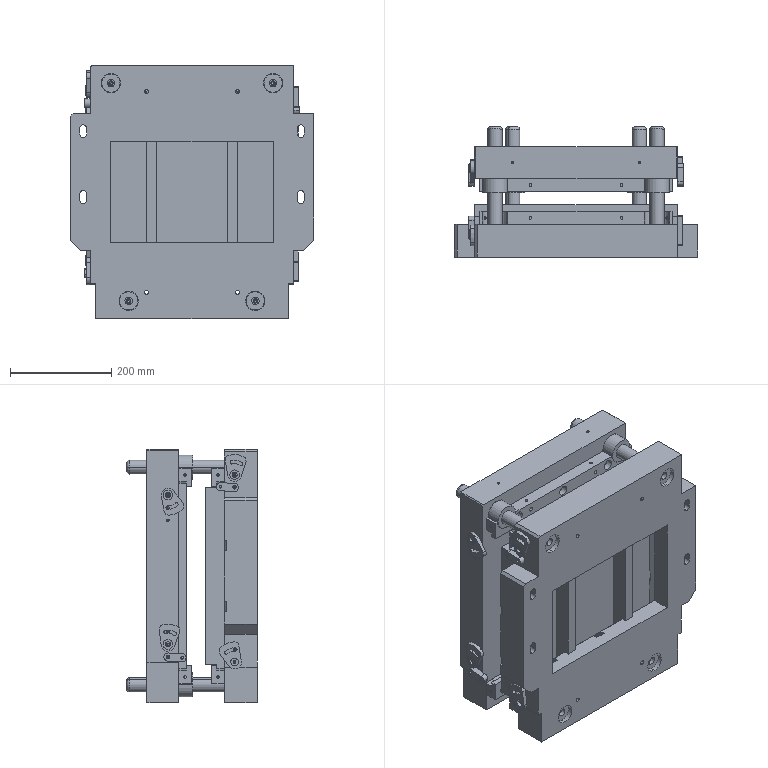Assembly | SolidWorks | mm | 38 component files | 38 solids | 988 faces | box 480 x 258 x 500 mm | volume 30255703 mm3 | cylinder 475 | plane 363 | cone 90 | torus 60 | commonest cylinder face diameters 5 x86 20 x44 48 x40 13.5 x36 8 x36 28 x32 38 x24 6.6 x24
Bill of materials:
MoldStopBlock001 | 4 |  | Flat plate with a tapered, rounded teardrop/trapezoid outline, one round through-hole near the narrow end and a curved arc slot near the wide end.
AdditionalStop | 3 |  | Thick block with a stadium/obround outline (link-like) and two round through-holes, one near each rounded end; one hole looks slightly larger than the other. A small step runs across the mid-length of one face.
GuideSlot1-01 | 2 |  | Long rectangular bar with two large semicircular saddle cutouts on the top edge near each end, a row of through-holes across the side face, small holes on the top face, and stepped/notched end blocks.
GuideSlot1 | 2 |  | Long rectangular bar with a stepped (rabbeted) L-shaped cross-section, two semicircular cutouts open to the bottom edge, and a row of through-holes in the side face. It looks like a counterpart to a similar saddle bar.
LocatingPin | 2 |  | Plain solid cylindrical rod with one end rounded/domed and the other end apparently flat.
GuidePin | 4 |  | Slender cylindrical pin with a thin integral collar near one end, a short stub past the collar, a small axial center hole/recess in the stub end, and a slightly rounded or chamfered opposite end.
LowerDieSet | 1 |  | Thick rectangular frame plate with a large central rectangular opening, stepped side tabs, chamfered corners, large corner holes, small holes, slotted holes on the side tabs, and small holes and notches on the edges.
MoldPlate | 1 |  | Plain rectangular plate with a small step or lip along two opposite edges, giving a slightly offset or rabbeted edge profile.
MoldSlotBaffle | 4 |  | Rectangular block or plate with four chamfered corners and two round through-holes lined up along one side of the face.
PinDiameter15 | 3 |  | Flanged cylindrical bushing: a thin wide flange on one end of a cylindrical body, with a straight central through-bore.
ReinforcingRib001 | 2 |  | Long narrow flat bar with chamfered corners at both ends and two small through-holes near the ends; the cross-section has bevelled long edges.
SpacerBlock | 4 |  | Stepped annular washer/spacer: a wider disc with a smaller-diameter raised boss on one side and a central through-hole.
GuideBushing | 4 |  | Hollow cylindrical sleeve (thick-walled tube) with a concentric through-bore and three narrow, round-bottomed circumferential grooves grouped near one end of the outer surface; the remaining length is plain.
KF525R2-MJ-A001 | 1 | 55 | Thick rectangular plate with a step: one end section is slightly narrower than the main body. It has four large through-holes near the corners, several small holes on the main face near each end, and small holes on the edge faces.
MoldUpperPlate510x280 | 1 |  | Plain thin rectangular plate or block with flat parallel faces and no visible holes, cutouts, or edge features.
Mates:
1. concentric | PinDiameter15-1 face at (-266.846, -14.073, 553) dir (1, 0, 0) r 7.5 | MoldStopBlock001-1 face at (-264.896, -14.073, 553) dir (1, 0, 0) r 7.5
2. coincident | PinDiameter15-1 face at (-264.896, -14.073, 553) dir (1, 0, 0) | MoldStopBlock001-1 face at (-264.896, -14.073, 553) dir (-1, 0, 0)
3. concentric | NewDieSet-1/LowerDieSetAssembly-1/LowerDieSet-1 face at (-256.746, -14.073, 553) dir (-1, 0, 0) r 2.5 | PinDiameter15-1 face at (-266.846, -14.073, 553) dir (-1, 0, 0) r 2.65
4. coincident | NewDieSet-1/LowerDieSetAssembly-1/LowerDieSet-1 face at (-256.746, -59.073, 603) dir (-1, 0, 0) | PinDiameter15-1 face at (-256.746, -14.073, 553) dir (1, 0, 0)
5. parallel | LowerDieSetAssembly-1/LowerDieSet-1 face at (329.721, -20.659, 572.489) dir (0, 1, 0) | UpperDieSetAssembly-1/KF525R2-MJ-A001-1 face at (-70.279, 69.341, 572.489) dir (0, -1, 0)
6. concentric | LowerDieSetAssembly-1/LowerDieSet-1 face at (254.721, -70.659, 107.489) dir (0, -1, 0) r 19 | SpacerBlock-1 face at (254.721, -77.659, 107.489) dir (0, 1, 0) r 18
7. coincident | SpacerBlock-2 face at (4.721, -77.659, 107.489) dir (0, -1, 0) | SpacerBlock-3 face at (-30.279, -77.659, 537.489) dir (0, -1, 0)
8. coincident | SpacerBlock-3 face at (-30.279, -77.659, 537.489) dir (0, -1, 0) | SpacerBlock-4 face at (289.721, -77.659, 537.489) dir (0, -1, 0)
9. coincident | SpacerBlock-1 face at (254.721, -77.659, 107.489) dir (0, -1, 0) | SpacerBlock-4 face at (289.721, -77.659, 537.489) dir (0, -1, 0)
10. coincident | LowerDieSetAssembly-1/LowerDieSet-1 face at (254.721, -70.659, 107.489) dir (0, -1, 0) | SpacerBlock-1 face at (254.721, -70.659, 107.489) dir (0, 1, 0)
11. concentric | LowerDieSetAssembly-1/LowerDieSet-1 face at (-30.279, -70.659, 537.489) dir (0, -1, 0) r 19 | SpacerBlock-3 face at (-30.279, -77.659, 537.489) dir (0, 1, 0) r 18
12. concentric | NewDieSet face at (59.721, 111.341, 32.489) dir (0, -1, 0) r 4 | LocatingPin-1 face at (39.721, 4.341, 520.589) dir (0, -1, 0) r 4
13. distance | LocatingPin-1 face at (39.721, 4.341, 520.589) dir (0, 1, 0) | NewDieSet face at (-0.2789, -20.659, 42.189) dir (0, -1, 0)
14. concentric | NewDieSet face at (139.721, 111.341, 32.489) dir (0, -1, 0) r 4 | LocatingPin-2 face at (219.721, 4.341, 520.589) dir (0, -1, 0) r 4
15. distance | NewDieSet face at (-0.2789, -20.659, 42.189) dir (0, -1, 0) | LocatingPin-2 face at (219.721, -35.659, 520.589) dir (0, -1, 0)
16. parallel | LowerDieSetAssembly-1/LowerDieSet-1 face at (329.721, -85.659, 572.489) dir (0, -1, 0) | NewDieSet plane at (0, 0, 0) dir (0, 1, 0)
17. concentric | LowerDieSetAssembly-1/GuidePin-4 face at (289.721, -47.659, 537.489) dir (0, -1, 0) r 3.4 | SpacerBlock-4 face at (289.721, -77.659, 537.489) dir (0, -1, 0) r 7.5
18. concentric | LowerDieSetAssembly-1/LowerDieSet-1 edge at (4.721, -70.659, 107.489) dir (0, -1, 0) r 19 | SpacerBlock-2 face at (4.721, -77.659, 107.489) dir (0, -1, 0) r 7.5
19. coincident | LocatingPin-1 face at (39.721, 4.341, 520.589) dir (0, 1, 0) | LocatingPin-2 face at (219.721, 4.341, 520.589) dir (0, 1, 0)
20. distance | LocatingPin-1 face at (39.721, -35.659, 520.589) dir (0, -1, 0) | LowerDieSetAssembly-1/LowerDieSet-1 face at (329.721, -20.659, 572.489) dir (0, 1, 0)
21. coincident | LowerDieSetAssembly-1/LowerDieSet-1 face at (329.721, -20.659, 572.489) dir (0, 1, 0) | GuideSlot1-01-4 face at (319.721, -20.659, 505.589) dir (0, -1, 0)
22. parallel | LowerDieSetAssembly-1/LowerDieSet-1 face at (329.721, -85.659, 572.489) dir (0, 0, 1) | GuideSlot1-01-4 face at (319.721, 4.441, 505.589) dir (0, 0, -1)
23. width | GuideSlot1-01-4 face at (-60.279, 4.441, 505.589) dir (-1, 0, 0) | GuideSlot1-01-4 face at (319.721, 4.441, 505.589) dir (1, 0, 0) | LowerDieSetAssembly-1/LowerDieSet-1 face at (-70.279, -85.659, 572.489) dir (-1, 0, 0) | LowerDieSetAssembly-1/LowerDieSet-1 face at (329.721, -85.659, 572.489) dir (1, 0, 0)
24. concentric | LowerDieSetAssembly-1/GuidePin-3 face at (-30.279, -47.659, 537.489) dir (0, 1, 0) r 14 | UpperDieSetAssembly-1/GuideBushing-1 face at (-30.279, 132.341, 537.489) dir (0, -1, 0) r 14
25. concentric | LowerDieSetAssembly-1/GuidePin-1 face at (254.721, -47.659, 107.489) dir (0, 1, 0) r 14 | UpperDieSetAssembly-1/GuideBushing-3 face at (254.721, 132.341, 107.489) dir (0, -1, 0) r 14
26. distance | UpperDieSetAssembly-1/KF525R2-MJ-A001-1 face at (-70.279, 69.341, 572.489) dir (0, -1, 0) | LowerDieSetAssembly-1/LowerDieSet-1 face at (329.721, -20.659, 572.489) dir (0, 1, 0)
27. concentric | LocatingPin-1 face at (39.721, 4.341, 520.589) dir (0, -1, 0) r 4 | GuideSlot1-01-4 face at (39.721, 111.341, 520.589) dir (0, -1, 0) r 4
28. concentric | LocatingPin-2 face at (219.721, 4.341, 520.589) dir (0, -1, 0) r 4 | GuideSlot1-01-4 face at (219.721, 111.341, 520.589) dir (0, -1, 0) r 4
29. parallel | LowerDieSetAssembly-1/LowerDieSet-1 face at (329.721, -85.659, 72.489) dir (0, 0, -1) | GuideSlot1-2 face at (-60.279, 4.441, 139.389) dir (0, 0, 1)
30. coincident | LowerDieSetAssembly-1/LowerDieSet-1 face at (329.721, -20.659, 572.489) dir (0, 1, 0) | GuideSlot1-2 face at (-60.279, -20.659, 139.389) dir (0, -1, 0)
31. coincident | LowerDieSetAssembly-1/LowerDieSet-1 face at (39.721, -59.659, 172.489) dir (1, 0, 0) | ReinforcingRib001-2 face at (39.721, -59.659, 472.489) dir (-1, 0, 0)
32. coincident | LowerDieSetAssembly-1/LowerDieSet-1 face at (59.721, -59.659, 472.489) dir (0, 0, -1) | ReinforcingRib001-2 face at (49.721, -40.159, 472.489) dir (0, 0, 1)
33. coincident | LowerDieSetAssembly-1/LowerDieSet-1 face at (329.721, -20.659, 572.489) dir (0, 1, 0) | ReinforcingRib001-2 face at (39.721, -20.659, 472.489) dir (0, 1, 0)
34. coincident | LowerDieSetAssembly-1/LowerDieSet-1 face at (329.721, -20.659, 572.489) dir (0, 1, 0) | ReinforcingRib001-1 face at (199.721, -20.659, 472.489) dir (0, 1, 0)
35. coincident | UpperDieSetAssembly-1/KF525R2-MJ-A001-1 face at (-70.279, 69.341, 572.489) dir (0, -1, 0) | GuideSlot1-01-5 face at (-60.279, 69.341, 505.589) dir (0, 1, 0)
36. coincident | UpperDieSetAssembly-1/KF525R2-MJ-A001-1 face at (-70.279, 69.341, 572.489) dir (0, -1, 0) | GuideSlot1-4 face at (319.721, 69.341, 139.389) dir (0, 1, 0)
37. concentric | UpperDieSetAssembly-1/KF525R2-MJ-A001-1 face at (294.721, 69.341, 124.389) dir (0, -1, 0) r 5.1 | GuideSlot1-4 face at (294.721, 44.241, 124.389) dir (0, -1, 0) r 10
38. concentric | UpperDieSetAssembly-1/KF525R2-MJ-A001-1 face at (-35.279, 69.341, 124.389) dir (0, -1, 0) r 5.1 | GuideSlot1-4 face at (-35.279, 44.241, 124.389) dir (0, -1, 0) r 10
39. parallel | UpperDieSetAssembly-1/KF525R2-MJ-A001-1 face at (-70.279, 132.341, 572.489) dir (0, 1, 0) | MoldSlotBaffle-6 face at (329.721, 54.341, 219.989) dir (0, -1, 0)
40. concentric | UpperDieSetAssembly-1/KF525R2-MJ-A001-1 face at (329.721, 90.841, 212.489) dir (1, 0, 0) r 2.5 | MoldSlotBaffle-6 face at (329.721, 90.841, 212.489) dir (-1, 0, 0) r 3.3
41. coincident | UpperDieSetAssembly-1/KF525R2-MJ-A001-1 face at (329.721, 132.341, 572.489) dir (1, 0, 0) | MoldSlotBaffle-6 face at (329.721, 54.341, 219.989) dir (-1, 0, 0)
42. parallel | LowerDieSetAssembly-1/LowerDieSet-1 face at (329.721, -40.659, 177.489) dir (1, 0, 0) r 2.5 | MoldSlotBaffle-7 face at (339.721, -40.659, 177.489) dir (1, 0, 0) r 3.3
43. coincident | LowerDieSetAssembly-1/LowerDieSet-1 face at (329.721, -85.659, 572.489) dir (1, 0, 0) | MoldSlotBaffle-7 face at (329.721, -4.159, 184.989) dir (-1, 0, 0)
44. concentric | LowerDieSetAssembly-1/LowerDieSet-1 face at (329.721, -40.659, 177.489) dir (1, 0, 0) r 2.5 | MoldSlotBaffle-7 face at (339.721, -40.659, 177.489) dir (1, 0, 0) r 3.3
45. concentric | UpperDieSetAssembly-1/KF525R2-MJ-A001-1 face at (329.721, 90.841, 457.489) dir (1, 0, 0) r 2.5 | MoldSlotBaffle-8 face at (329.721, 90.841, 457.489) dir (-1, 0, 0) r 3.3
46. coincident | UpperDieSetAssembly-1/KF525R2-MJ-A001-1 face at (329.721, 132.341, 572.489) dir (1, 0, 0) | MoldSlotBaffle-8 face at (329.721, 54.341, 464.989) dir (-1, 0, 0)
47. concentric | UpperDieSetAssembly-1/KF525R2-MJ-A001-1 face at (329.721, 90.841, 432.489) dir (1, 0, 0) r 2.5 | MoldSlotBaffle-8 face at (329.721, 90.841, 432.489) dir (-1, 0, 0) r 3.3
48. coincident | UpperDieSetAssembly-1/KF525R2-MJ-A001-1 face at (-70.279, 132.341, 572.489) dir (-1, 0, 0) | MoldStopBlock001-1 face at (-70.279, 90.841, 187.489) dir (1, 0, 0)
49. coincident | UpperDieSetAssembly-1/KF525R2-MJ-A001-1 face at (-70.279, 132.341, 572.489) dir (-1, 0, 0) | PinDiameter15-3 face at (-70.279, 90.841, 187.489) dir (1, 0, 0)
50. concentric | UpperDieSetAssembly-1/KF525R2-MJ-A001-1 face at (-70.279, 90.841, 482.489) dir (-1, 0, 0) r 2.5 | MoldStopBlock001-6 face at (-78.279, 90.841, 482.489) dir (1, 0, 0) r 7.5
51. coincident | UpperDieSetAssembly-1/KF525R2-MJ-A001-1 face at (-70.279, 132.341, 572.489) dir (-1, 0, 0) | MoldStopBlock001-6 face at (-70.279, 90.841, 482.489) dir (1, 0, 0)
52. concentric | MoldStopBlock001-6 face at (-78.279, 90.841, 482.489) dir (1, 0, 0) r 7.5 | PinDiameter15-5 face at (-80.379, 90.841, 482.489) dir (1, 0, 0) r 7.5
53. coincident | UpperDieSetAssembly-1/KF525R2-MJ-A001-1 face at (-70.279, 132.341, 572.489) dir (-1, 0, 0) | PinDiameter15-5 face at (-70.279, 90.841, 482.489) dir (1, 0, 0)
54. concentric | MoldStopBlock001-1 face at (-78.279, 90.841, 187.489) dir (1, 0, 0) r 7.5 | PinDiameter15-3 face at (-80.379, 90.841, 187.489) dir (-1, 0, 0) r 2.65
55. concentric | UpperDieSetAssembly-1/KF525R2-MJ-A001-1 face at (-70.279, 90.841, 187.489) dir (-1, 0, 0) r 2.5 | PinDiameter15-3 face at (-80.379, 90.841, 187.489) dir (-1, 0, 0) r 2.65
56. concentric | LowerDieSetAssembly-1/LowerDieSet-1 face at (254.721, -20.659, 520.589) dir (0, 1, 0) r 5.1 | GuideSlot1-01-4 face at (254.721, 4.441, 520.589) dir (0, 1, 0) r 10
57. concentric | LowerDieSetAssembly-1/LowerDieSet-1 face at (-70.279, -40.659, 152.489) dir (-1, 0, 0) r 2.5 | MoldStopBlock001-7 face at (-78.279, -40.659, 152.489) dir (1, 0, 0) r 7.5
58. coincident | LowerDieSetAssembly-1/LowerDieSet-1 face at (-70.279, -85.659, 572.489) dir (-1, 0, 0) | MoldStopBlock001-7 face at (-70.279, -40.659, 152.489) dir (1, 0, 0)
59. concentric | LowerDieSetAssembly-1/LowerDieSet-1 face at (329.721, -40.659, 497.489) dir (1, 0, 0) r 2.5 | MoldSlotBaffle-9 face at (339.721, -40.659, 497.489) dir (1, 0, 0) r 3.3
60. concentric | LowerDieSetAssembly-1/LowerDieSet-1 face at (329.721, -40.659, 522.489) dir (1, 0, 0) r 2.5 | MoldSlotBaffle-9 face at (339.721, -40.659, 522.489) dir (1, 0, 0) r 3.3
61. coincident | LowerDieSetAssembly-1/LowerDieSet-1 face at (329.721, -85.659, 572.489) dir (1, 0, 0) | MoldSlotBaffle-9 face at (329.721, -4.159, 529.989) dir (-1, 0, 0)
62. coincident | LowerDieSetAssembly-1/LowerDieSet-1 face at (-70.279, -85.659, 572.489) dir (-1, 0, 0) | AdditionalStop-1 face at (-70.279, -40.659, 497.489) dir (1, 0, 0)
63. concentric | LowerDieSetAssembly-1/LowerDieSet-1 face at (-70.279, -40.659, 497.489) dir (-1, 0, 0) r 2.5 | AdditionalStop-1 face at (-70.279, -40.659, 497.489) dir (-1, 0, 0) r 3.25
64. coincident | UpperDieSetAssembly-1/KF525R2-MJ-A001-1 face at (-70.279, 132.341, 572.489) dir (-1, 0, 0) | AdditionalStop-2 face at (-70.279, 90.841, 162.489) dir (1, 0, 0)
65. concentric | UpperDieSetAssembly-1/KF525R2-MJ-A001-1 face at (-70.279, 90.841, 162.489) dir (-1, 0, 0) r 2.5 | AdditionalStop-2 face at (-70.279, 90.841, 162.489) dir (-1, 0, 0) r 3.25
66. coincident | UpperDieSetAssembly-1/KF525R2-MJ-A001-1 face at (329.721, 132.341, 572.489) dir (1, 0, 0) | AdditionalStop-3 face at (329.721, 90.841, 482.489) dir (-1, 0, 0)
67. concentric | UpperDieSetAssembly-1/KF525R2-MJ-A001-1 face at (329.721, 90.841, 482.489) dir (1, 0, 0) r 2.5 | AdditionalStop-3 face at (329.721, 90.841, 482.489) dir (1, 0, 0) r 3.25
68. concentric | LowerDieSet-1 face at (-190.542, -34.836, 195) dir (0, 1, 0) r 14 | GuidePin-1 face at (-190.542, -7.836, 195) dir (0, -1, 0) r 14
69. coincident | GuidePin-3 face at (94.458, -227.836, 625) dir (0, -1, 0) | GuidePin-4 face at (-225.542, -227.836, 625) dir (0, -1, 0)
70. coincident | GuidePin-2 face at (59.458, -227.836, 195) dir (0, -1, 0) | GuidePin-3 face at (94.458, -227.836, 625) dir (0, -1, 0)
71. coincident | GuidePin-1 face at (-190.542, -227.836, 195) dir (0, -1, 0) | GuidePin-2 face at (59.458, -227.836, 195) dir (0, -1, 0)
72. concentric | LowerDieSet-1 face at (59.458, -34.836, 195) dir (0, 1, 0) r 14 | GuidePin-2 face at (59.458, -7.836, 195) dir (0, -1, 0) r 14
73. concentric | LowerDieSet-1 face at (94.458, -34.836, 625) dir (0, 1, 0) r 14 | GuidePin-3 face at (94.458, -7.836, 625) dir (0, -1, 0) r 14
74. concentric | LowerDieSet-1 face at (-225.542, -34.836, 625) dir (0, 1, 0) r 14 | GuidePin-4 face at (-225.542, -7.836, 625) dir (0, -1, 0) r 14
75. coincident | LowerDieSet-1 face at (-190.542, -26.836, 195) dir (0, -1, 0) | GuidePin-1 face at (-190.542, -26.836, 195) dir (0, 1, 0)
76. width | LowerDieSet-1 face at (-265.542, 30.164, 660) dir (-1, 0, 0) | LowerDieSet-1 face at (134.458, 30.164, 660) dir (1, 0, 0) | MoldPlate-1 face at (-265.542, -34.836, 593) dir (-1, 0, 0) | MoldPlate-1 face at (134.458, -34.836, 593) dir (1, 0, 0)
77. coincident | LowerDieSet-1 face at (-265.542, -34.836, 660) dir (0, -1, 0) | MoldPlate-1 face at (-265.542, -34.836, 593) dir (0, 1, 0)
78. width | LowerDieSet-1 face at (-265.542, 30.164, 660) dir (0, 0, 1) | LowerDieSet-1 face at (-265.542, 30.164, 160) dir (0, 0, -1) | MoldPlate-1 face at (-265.542, -34.836, 593) dir (0, 0, 1) | MoldPlate-1 face at (-265.542, -34.836, 227) dir (0, 0, -1)
79. width | LowerDieSet-1 face at (-265.542, 30.164, 660) dir (0, 0, 1) | LowerDieSet-1 face at (-265.542, 30.164, 160) dir (0, 0, -1) | MoldPlate-1 face at (-265.542, -34.836, 593) dir (0, 0, 1) | MoldPlate-1 face at (-265.542, -34.836, 227) dir (0, 0, -1)
80. concentric | KF525R2-MJ-A001-1 face at (-254.523, 30.027, 625) dir (0, 1, 0) r 24 | GuideBushing-1 face at (-254.523, 48.027, 625) dir (0, 1, 0) r 24
81. concentric | KF525R2-MJ-A001-1 face at (-219.523, 30.027, 195) dir (0, 1, 0) r 24 | GuideBushing-2 face at (-219.523, 48.027, 195) dir (0, 1, 0) r 24
82. coincident | GuideBushing-1 face at (-254.523, 3.027, 625) dir (0, -1, 0) | GuideBushing-2 face at (-219.523, 3.027, 195) dir (0, -1, 0)
83. concentric | KF525R2-MJ-A001-1 face at (65.477, 30.027, 625) dir (0, 1, 0) r 24 | GuideBushing-4 face at (65.477, 48.027, 625) dir (0, 1, 0) r 24
84. concentric | KF525R2-MJ-A001-1 face at (30.477, 30.027, 195) dir (0, 1, 0) r 24 | GuideBushing-3 face at (30.477, 48.027, 195) dir (0, 1, 0) r 24
85. coincident | GuideBushing-3 face at (30.477, 93.027, 195) dir (0, 1, 0) | GuideBushing-4 face at (65.477, 93.027, 625) dir (0, 1, 0)
86. coincident | KF525R2-MJ-A001-1 face at (-294.523, 93.027, 660) dir (0, 1, 0) | GuideBushing-1 face at (-254.523, 93.027, 625) dir (0, 1, 0)
87. coincident | KF525R2-MJ-A001-1 face at (-294.523, 93.027, 660) dir (0, 1, 0) | GuideBushing-3 face at (30.477, 93.027, 195) dir (0, 1, 0)
88. coincident | KF525R2-MJ-A001-1 face at (-294.523, 30.027, 660) dir (0, -1, 0) | MoldUpperPlate510x280-1 face at (-194.523, 30.027, 593) dir (0, 1, 0)
89. width | KF525R2-MJ-A001-1 face at (-294.523, 93.027, 160) dir (0, 0, -1) | KF525R2-MJ-A001-1 face at (-294.523, 93.027, 660) dir (0, 0, 1) | MoldUpperPlate510x280-1 face at (-194.523, 30.027, 227) dir (0, 0, -1) | MoldUpperPlate510x280-1 face at (-194.523, 30.027, 593) dir (0, 0, 1)
90. width | KF525R2-MJ-A001-1 face at (-294.523, 93.027, 660) dir (-1, 0, 0) | KF525R2-MJ-A001-1 face at (105.477, 93.027, 660) dir (1, 0, 0) | MoldUpperPlate510x280-1 face at (-194.523, 30.027, 593) dir (-1, 0, 0) | MoldUpperPlate510x280-1 face at (5.477, 30.027, 593) dir (1, 0, 0)